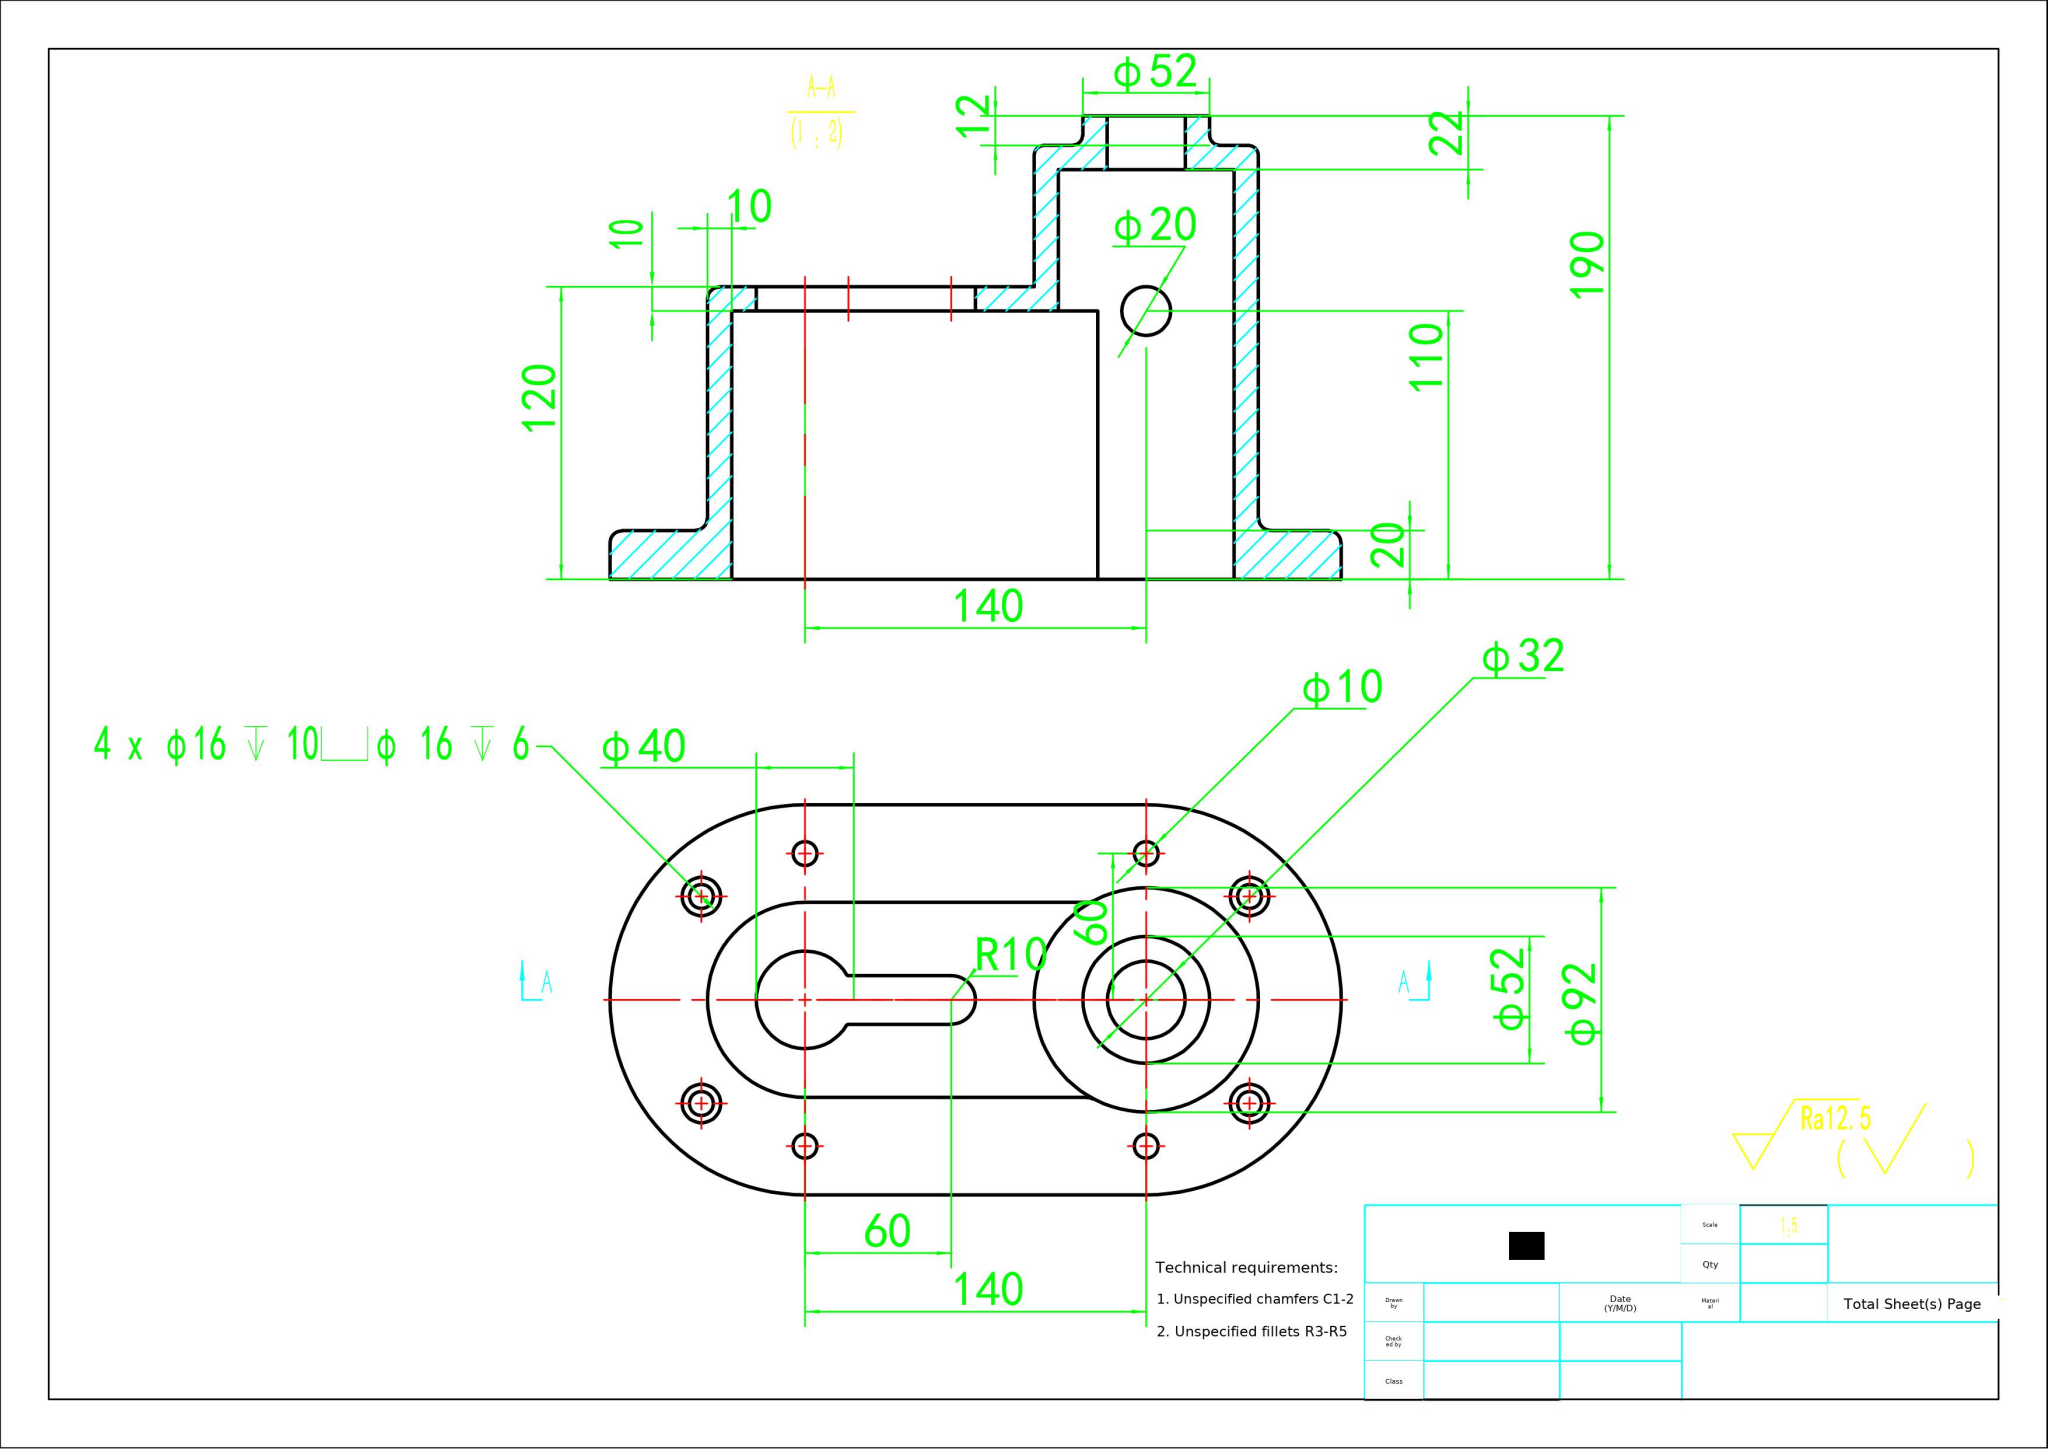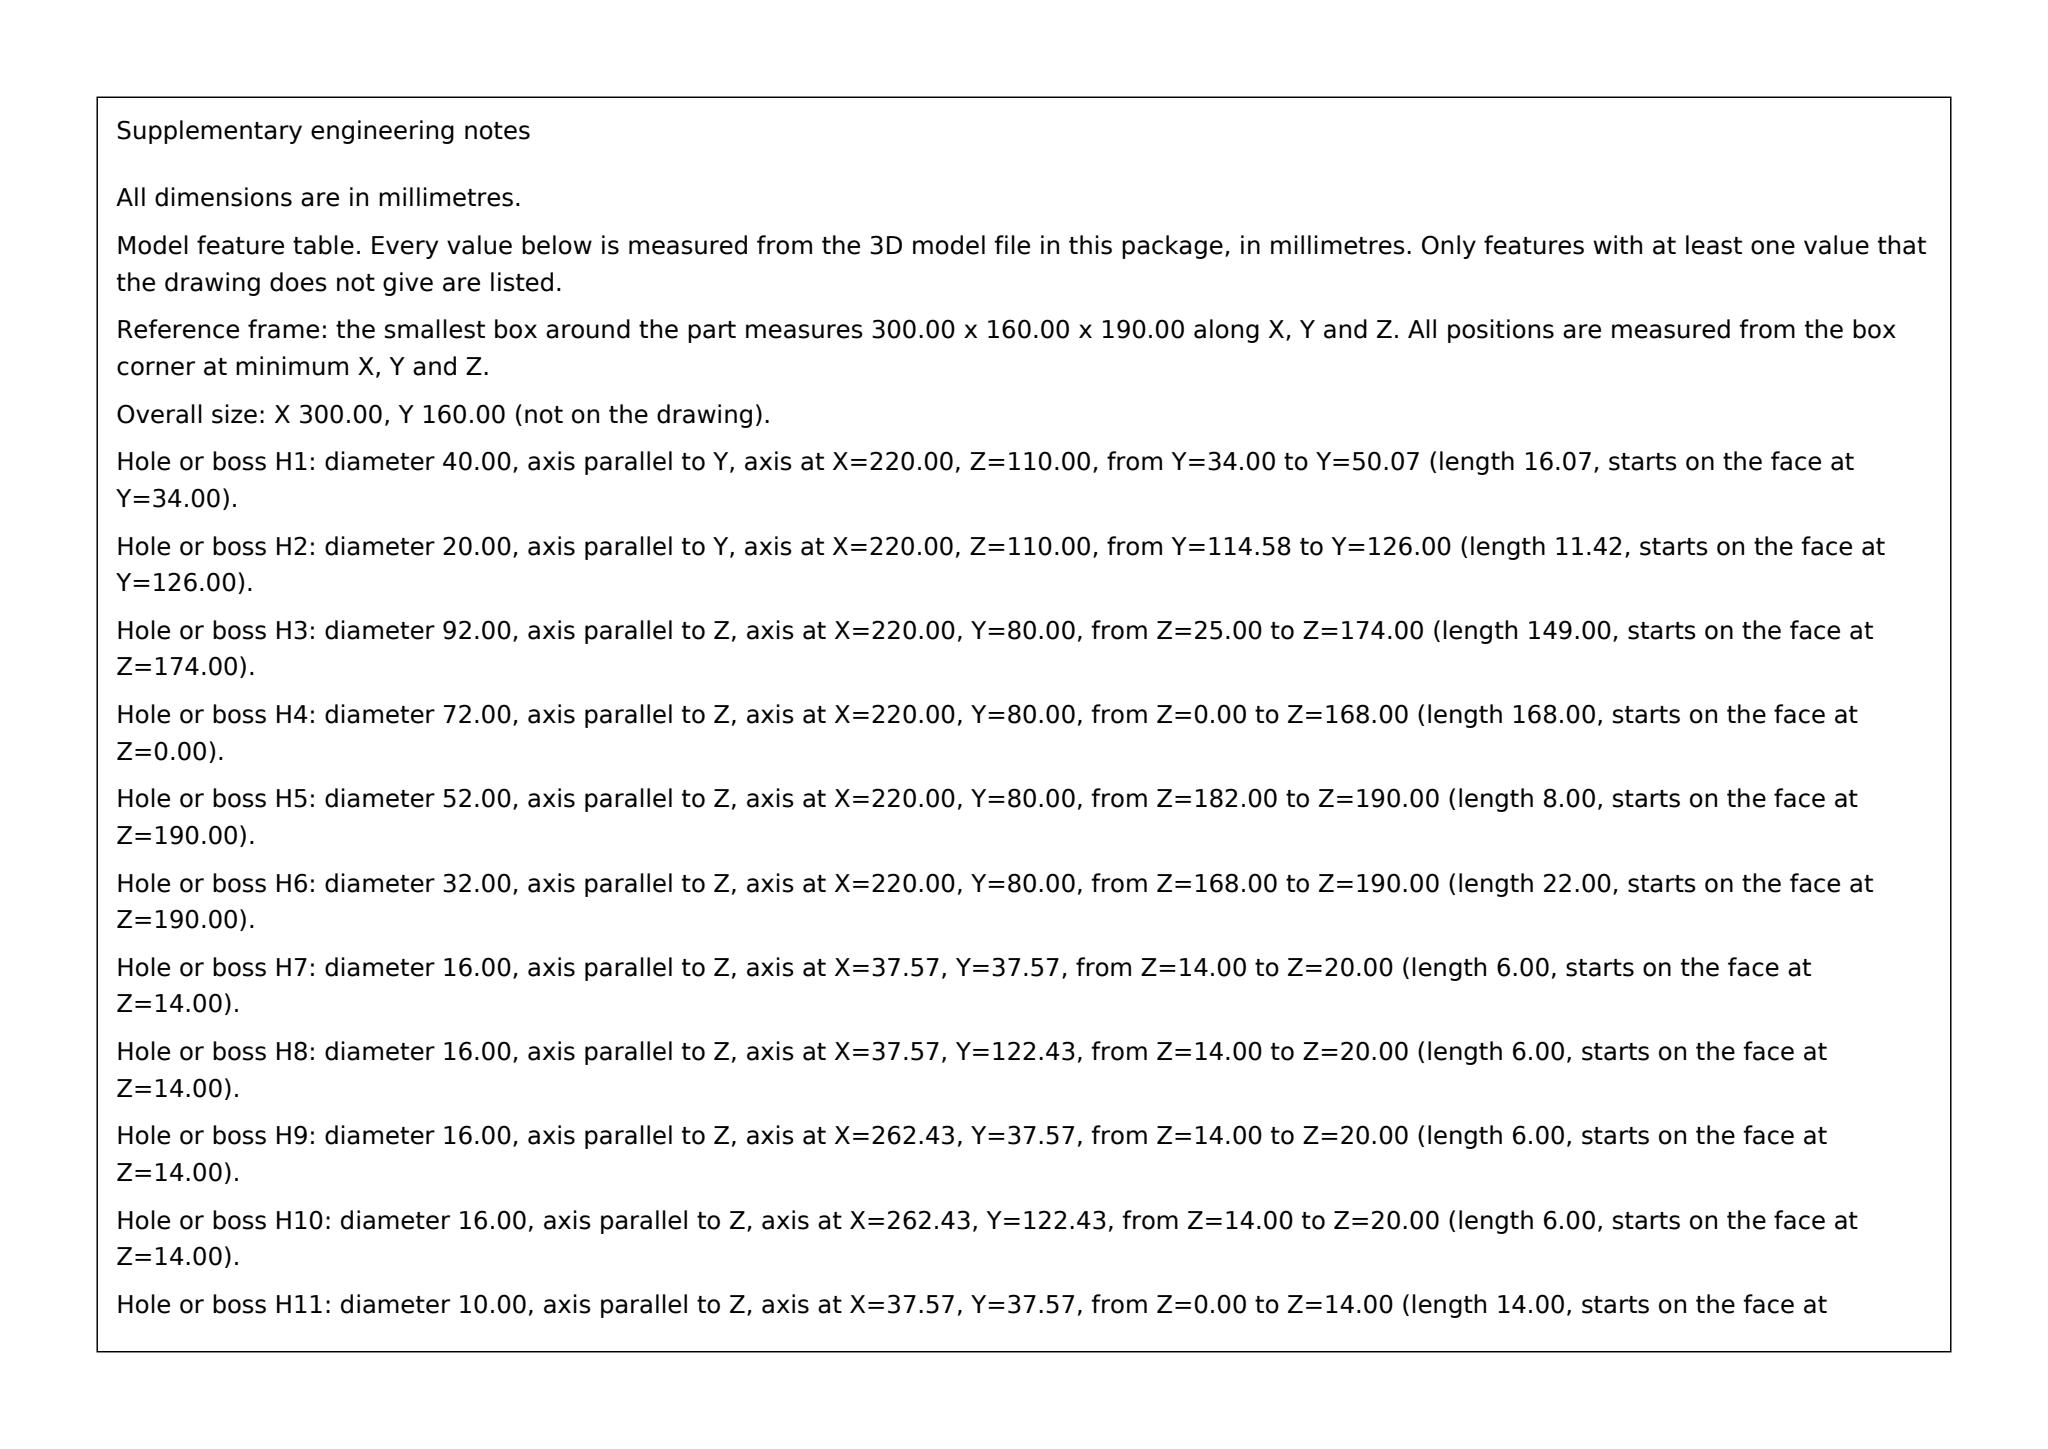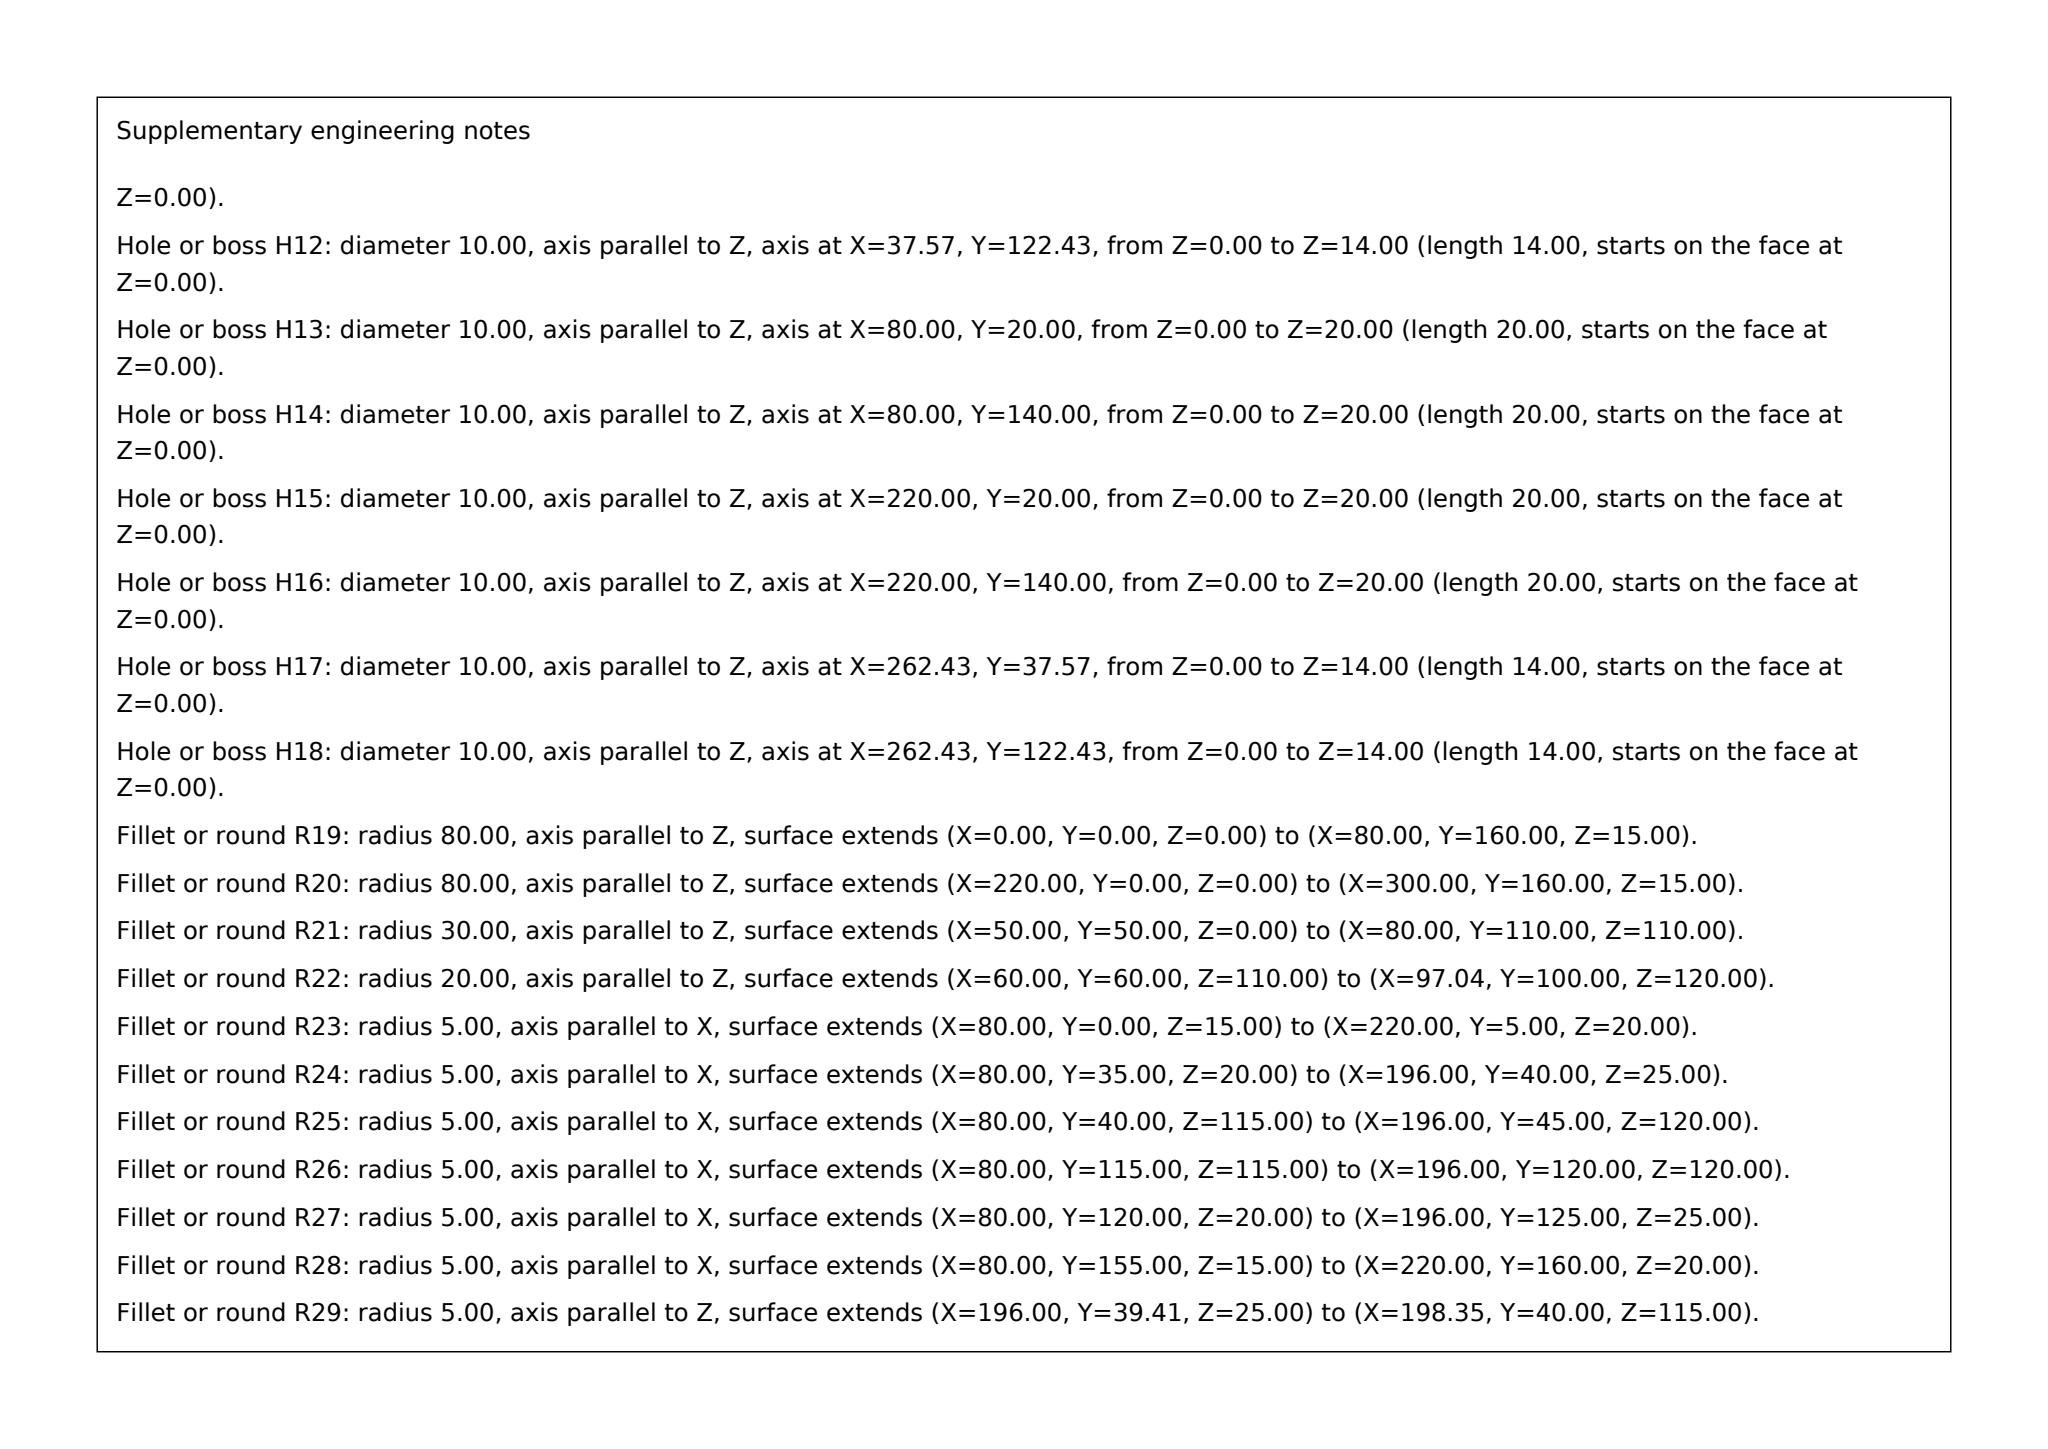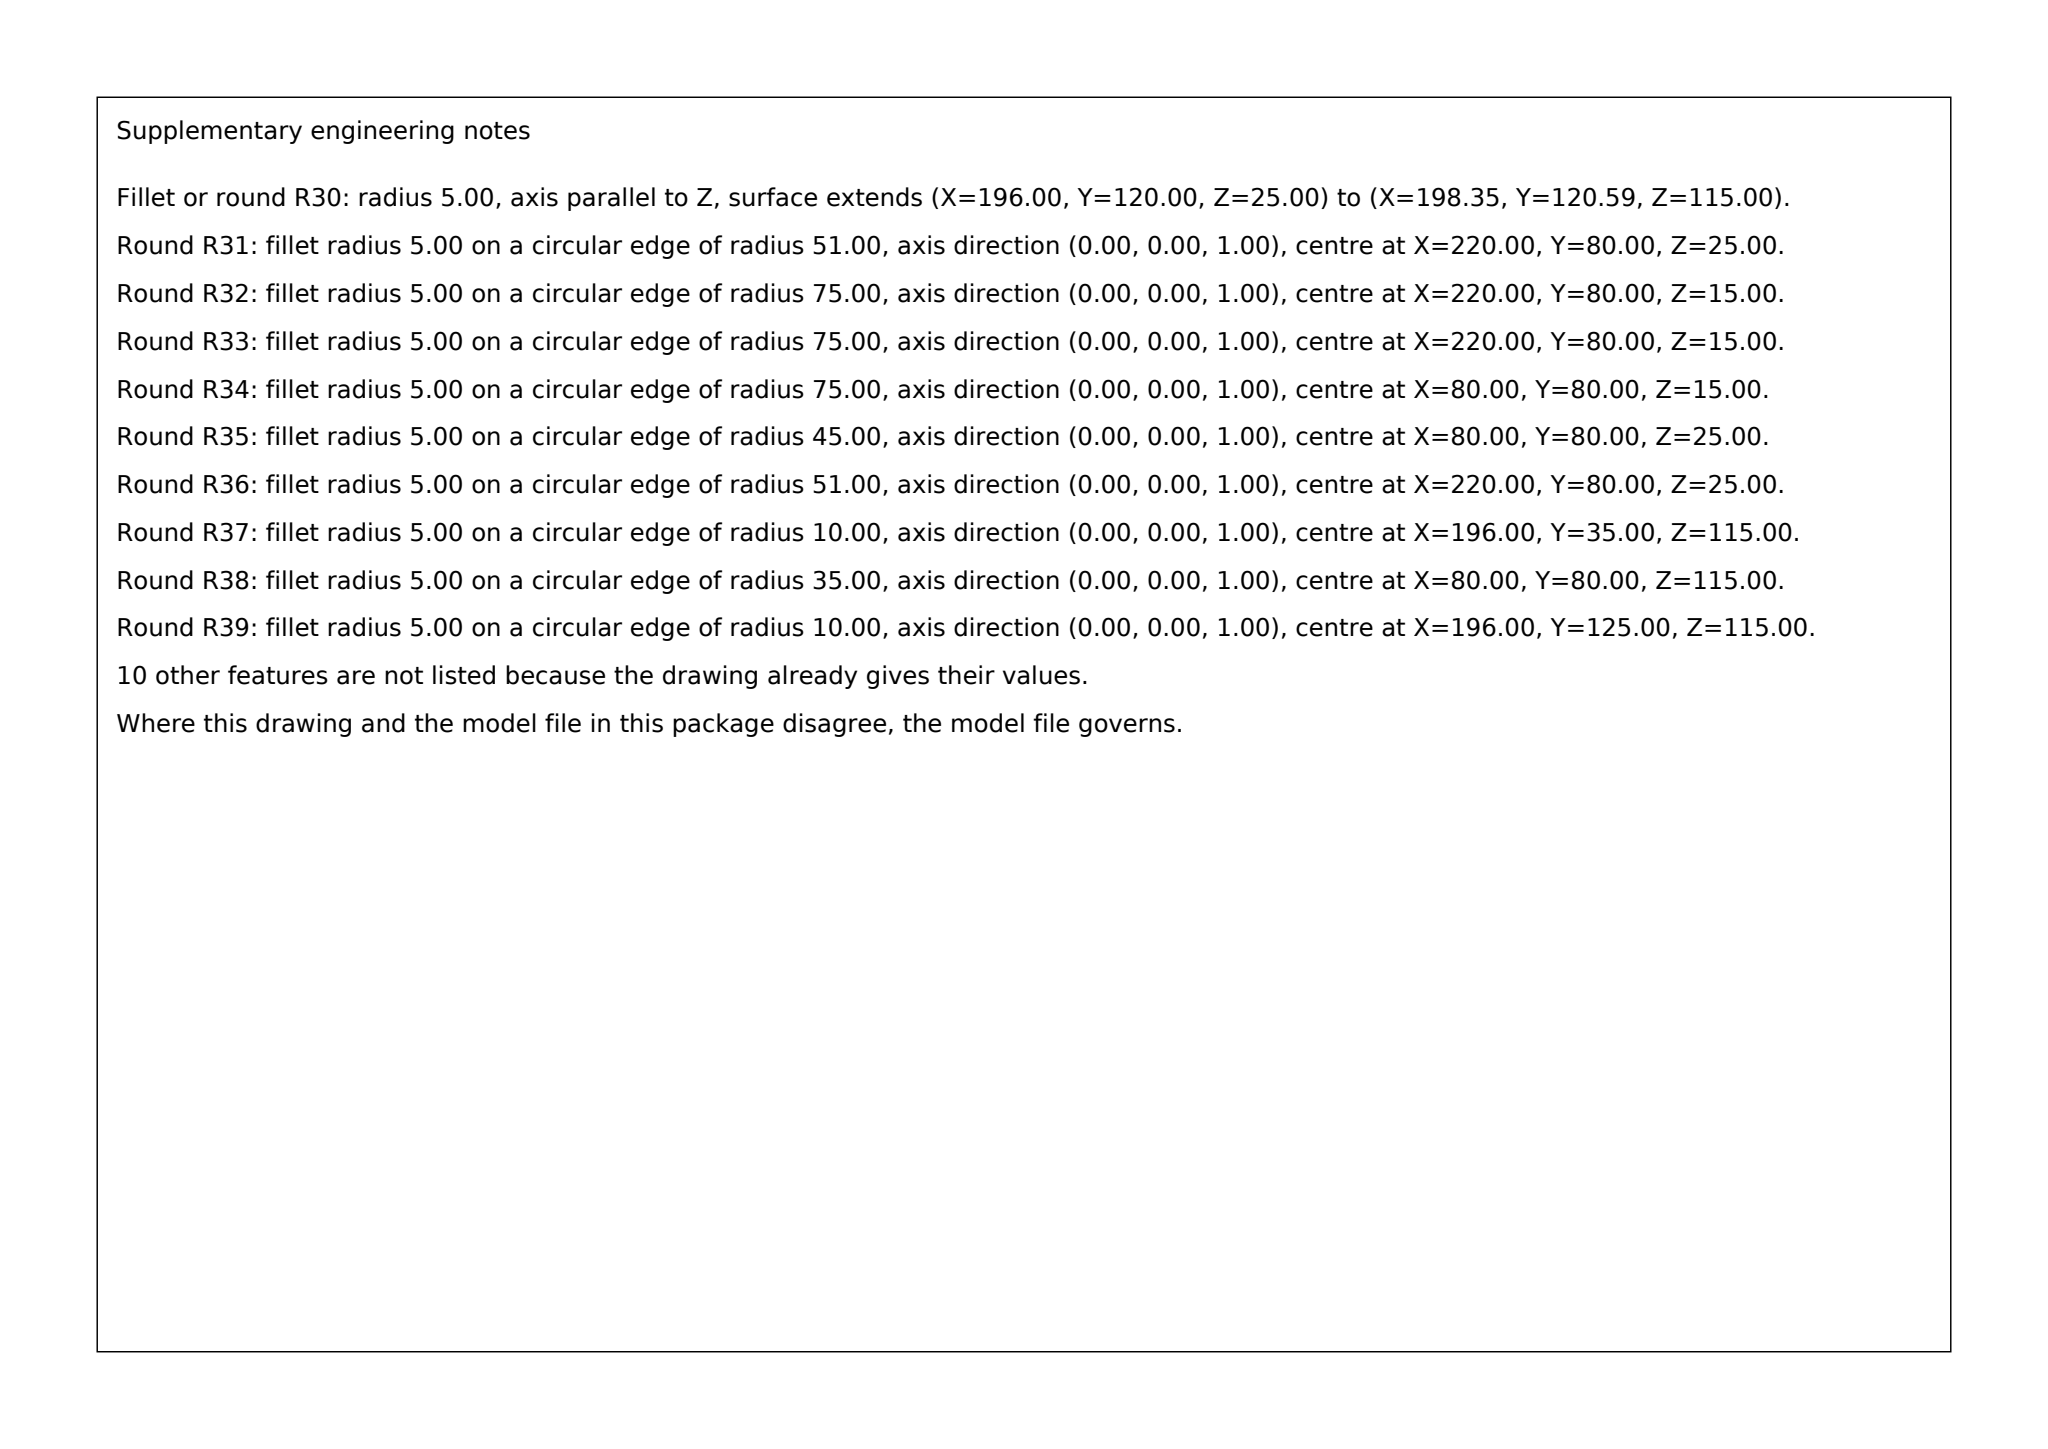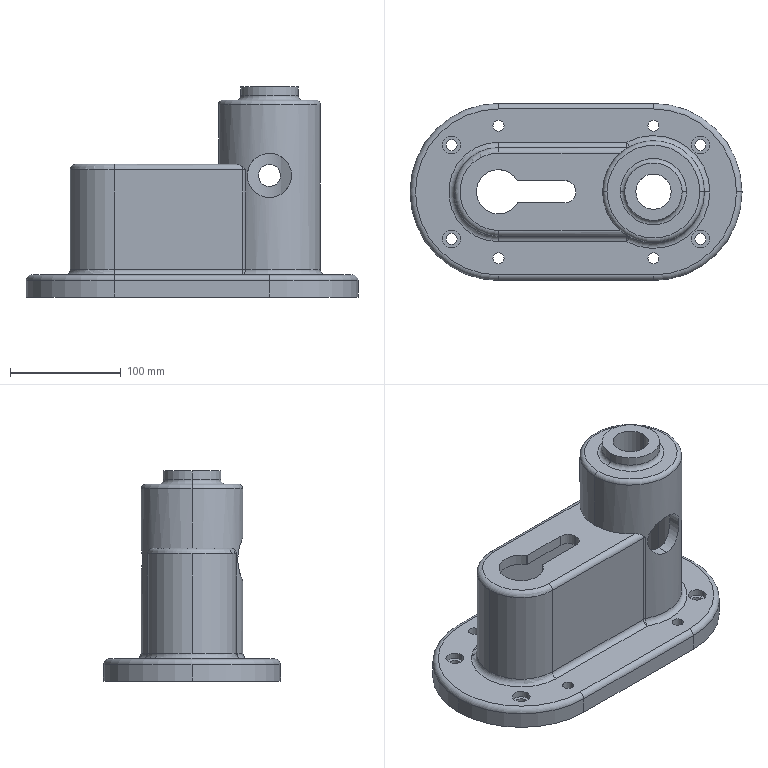Part | SolidWorks | mm | 1 solid | 89 faces | box 300 x 160 x 190 mm | volume 1350811 mm3 | cylinder 55 | plane 19 | torus 13 | sphere 2 | commonest cylinder face diameters 10 x24 16 x8 20 x4 40 x3 160 x3 72 x2 32 x2 52 x2